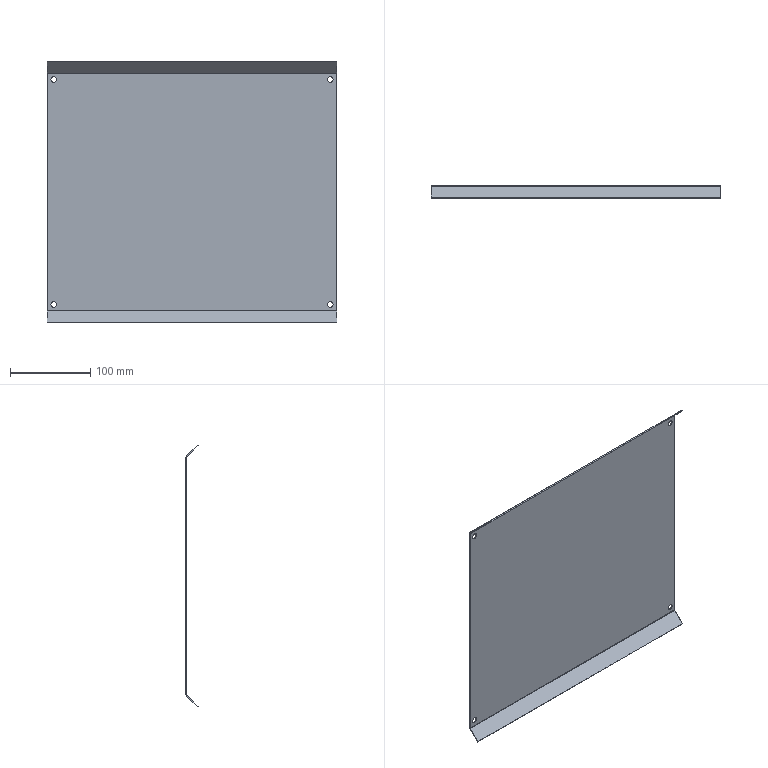Component | SolidWorks | CCD15ChainCover-1 | 1 solid | 30 faces | box 360 x 14.99 x 325.88 mm | volume 145179 mm3 | plane 18 | cylinder 12 | commonest cylinder face diameters 7 x8 3.873 x2 1.473 x2
STEP:
#1=CARTESIAN_POINT('',(-11.245,5.6,6.496));
#2=VERTEX_POINT('',#1);
#3=CARTESIAN_POINT('',(-11.521,5.6,6.496));
#4=VERTEX_POINT('',#3);
#5=CARTESIAN_POINT('',(-11.383,5.6,6.496));
#6=DIRECTION('',(0.,-1.,-0.));
#7=DIRECTION('',(-1.,-0.,-0.));
#8=AXIS2_PLACEMENT_3D('',#5,#6,#7);
#9=CIRCLE('',#8,0.1378);
#10=EDGE_CURVE('',#2,#4,#9,.T.);
#11=ORIENTED_EDGE('',*,*,#10,.T.);
#12=CARTESIAN_POINT('',(-11.521,5.648,6.496));
#13=VERTEX_POINT('',#12);
#14=CARTESIAN_POINT('',(-11.521,5.254,6.496));
#15=DIRECTION('',(-0.,1.,0.));
#16=VECTOR('',#15,39.37);
#17=LINE('',#14,#16);
#18=EDGE_CURVE('',#4,#13,#17,.T.);
#19=ORIENTED_EDGE('',*,*,#18,.T.);
#20=CARTESIAN_POINT('',(-11.245,5.648,6.496));
#21=VERTEX_POINT('',#20);
#22=CARTESIAN_POINT('',(-11.383,5.648,6.496));
#23=DIRECTION('',(-0.,1.,0.));
#24=DIRECTION('',(1.,0.,0.));
#25=AXIS2_PLACEMENT_3D('',#22,#23,#24);
#26=CIRCLE('',#25,0.1378);
#27=EDGE_CURVE('',#13,#21,#26,.T.);
#28=ORIENTED_EDGE('',*,*,#27,.T.);
#29=CARTESIAN_POINT('',(-11.245,5.254,6.496));
#30=DIRECTION('',(-0.,1.,0.));
#31=VECTOR('',#30,39.37);
#32=LINE('',#29,#31);
#33=EDGE_CURVE('',#2,#21,#32,.T.);
#34=ORIENTED_EDGE('',*,*,#33,.F.);
#35=EDGE_LOOP('',(#11,#19,#28,#34));
#36=FACE_OUTER_BOUND('',#35,.T.);
#37=CARTESIAN_POINT('',(-11.383,5.254,6.496));
#38=DIRECTION('',(-0.,1.,0.));
#39=DIRECTION('',(1.,0.,0.));
#40=AXIS2_PLACEMENT_3D('',#37,#38,#39);
#41=CYLINDRICAL_SURFACE('',#40,0.1378);
#42=ADVANCED_FACE('',(#36),#41,.F.);
#43=CARTESIAN_POINT('',(2.298,5.6,6.496));
#44=VERTEX_POINT('',#43);
#45=CARTESIAN_POINT('',(2.023,5.6,6.496));
#46=VERTEX_POINT('',#45);
#47=CARTESIAN_POINT('',(2.161,5.6,6.496));
#48=DIRECTION('',(0.,-1.,-0.));
#49=DIRECTION('',(-1.,-0.,-0.));
#50=AXIS2_PLACEMENT_3D('',#47,#48,#49);
#51=CIRCLE('',#50,0.1378);
#52=EDGE_CURVE('',#44,#46,#51,.T.);
#53=ORIENTED_EDGE('',*,*,#52,.T.);
#54=CARTESIAN_POINT('',(2.023,5.648,6.496));
#55=VERTEX_POINT('',#54);
#56=CARTESIAN_POINT('',(2.023,5.254,6.496));
#57=DIRECTION('',(-0.,1.,0.));
#58=VECTOR('',#57,39.37);
#59=LINE('',#56,#58);
#60=EDGE_CURVE('',#46,#55,#59,.T.);
#61=ORIENTED_EDGE('',*,*,#60,.T.);
#62=CARTESIAN_POINT('',(2.298,5.648,6.496));
#63=VERTEX_POINT('',#62);
#64=CARTESIAN_POINT('',(2.161,5.648,6.496));
#65=DIRECTION('',(-0.,1.,0.));
#66=DIRECTION('',(1.,0.,0.));
#67=AXIS2_PLACEMENT_3D('',#64,#65,#66);
#68=CIRCLE('',#67,0.1378);
#69=EDGE_CURVE('',#55,#63,#68,.T.);
#70=ORIENTED_EDGE('',*,*,#69,.T.);
#71=CARTESIAN_POINT('',(2.298,5.254,6.496));
#72=DIRECTION('',(-0.,1.,0.));
#73=VECTOR('',#72,39.37);
#74=LINE('',#71,#73);
#75=EDGE_CURVE('',#44,#63,#74,.T.);
#76=ORIENTED_EDGE('',*,*,#75,.F.);
#77=EDGE_LOOP('',(#53,#61,#70,#76));
#78=FACE_OUTER_BOUND('',#77,.T.);
#79=CARTESIAN_POINT('',(2.161,5.254,6.496));
#80=DIRECTION('',(-0.,1.,0.));
#81=DIRECTION('',(1.,0.,0.));
#82=AXIS2_PLACEMENT_3D('',#79,#80,#81);
#83=CYLINDRICAL_SURFACE('',#82,0.1378);
#84=ADVANCED_FACE('',(#78),#83,.F.);
#85=CARTESIAN_POINT('',(2.298,5.6,-4.528));
#86=VERTEX_POINT('',#85);
#87=CARTESIAN_POINT('',(2.023,5.6,-4.528));
#88=VERTEX_POINT('',#87);
#89=CARTESIAN_POINT('',(2.161,5.6,-4.528));
#90=DIRECTION('',(0.,-1.,-0.));
#91=DIRECTION('',(-1.,-0.,-0.));
#92=AXIS2_PLACEMENT_3D('',#89,#90,#91);
#93=CIRCLE('',#92,0.1378);
#94=EDGE_CURVE('',#86,#88,#93,.T.);
#95=ORIENTED_EDGE('',*,*,#94,.T.);
#96=CARTESIAN_POINT('',(2.023,5.648,-4.528));
#97=VERTEX_POINT('',#96);
#98=CARTESIAN_POINT('',(2.023,5.254,-4.528));
#99=DIRECTION('',(-0.,1.,0.));
#100=VECTOR('',#99,39.37);
#101=LINE('',#98,#100);
#102=EDGE_CURVE('',#88,#97,#101,.T.);
#103=ORIENTED_EDGE('',*,*,#102,.T.);
#104=CARTESIAN_POINT('',(2.298,5.648,-4.528));
#105=VERTEX_POINT('',#104);
#106=CARTESIAN_POINT('',(2.161,5.648,-4.528));
#107=DIRECTION('',(-0.,1.,0.));
#108=DIRECTION('',(1.,0.,0.));
#109=AXIS2_PLACEMENT_3D('',#106,#107,#108);
#110=CIRCLE('',#109,0.1378);
#111=EDGE_CURVE('',#97,#105,#110,.T.);
#112=ORIENTED_EDGE('',*,*,#111,.T.);
#113=CARTESIAN_POINT('',(2.298,5.254,-4.528));
#114=DIRECTION('',(-0.,1.,0.));
#115=VECTOR('',#114,39.37);
#116=LINE('',#113,#115);
#117=EDGE_CURVE('',#86,#105,#116,.T.);
#118=ORIENTED_EDGE('',*,*,#117,.F.);
#119=EDGE_LOOP('',(#95,#103,#112,#118));
#120=FACE_OUTER_BOUND('',#119,.T.);
#121=CARTESIAN_POINT('',(2.161,5.254,-4.528));
#122=DIRECTION('',(-0.,1.,0.));
#123=DIRECTION('',(1.,0.,0.));
#124=AXIS2_PLACEMENT_3D('',#121,#122,#123);
#125=CYLINDRICAL_SURFACE('',#124,0.1378);
#126=ADVANCED_FACE('',(#120),#125,.F.);
#127=CARTESIAN_POINT('',(-11.245,5.6,-4.528));
#128=VERTEX_POINT('',#127);
#129=CARTESIAN_POINT('',(-11.521,5.6,-4.528));
#130=VERTEX_POINT('',#129);
#131=CARTESIAN_POINT('',(-11.383,5.6,-4.528));
#132=DIRECTION('',(0.,-1.,-0.));
#133=DIRECTION('',(-1.,-0.,-0.));
#134=AXIS2_PLACEMENT_3D('',#131,#132,#133);
#135=CIRCLE('',#134,0.1378);
#136=EDGE_CURVE('',#128,#130,#135,.T.);
#137=ORIENTED_EDGE('',*,*,#136,.T.);
#138=CARTESIAN_POINT('',(-11.521,5.648,-4.528));
#139=VERTEX_POINT('',#138);
#140=CARTESIAN_POINT('',(-11.521,5.254,-4.528));
#141=DIRECTION('',(-0.,1.,0.));
#142=VECTOR('',#141,39.37);
#143=LINE('',#140,#142);
#144=EDGE_CURVE('',#130,#139,#143,.T.);
#145=ORIENTED_EDGE('',*,*,#144,.T.);
#146=CARTESIAN_POINT('',(-11.245,5.648,-4.528));
#147=VERTEX_POINT('',#146);
#148=CARTESIAN_POINT('',(-11.383,5.648,-4.528));
#149=DIRECTION('',(-0.,1.,0.));
#150=DIRECTION('',(1.,0.,0.));
#151=AXIS2_PLACEMENT_3D('',#148,#149,#150);
#152=CIRCLE('',#151,0.1378);
#153=EDGE_CURVE('',#139,#147,#152,.T.);
#154=ORIENTED_EDGE('',*,*,#153,.T.);
#155=CARTESIAN_POINT('',(-11.245,5.254,-4.528));
#156=DIRECTION('',(-0.,1.,0.));
#157=VECTOR('',#156,39.37);
#158=LINE('',#155,#157);
#159=EDGE_CURVE('',#128,#147,#158,.T.);
#160=ORIENTED_EDGE('',*,*,#159,.F.);
#161=EDGE_LOOP('',(#137,#145,#154,#160));
#162=FACE_OUTER_BOUND('',#161,.T.);
#163=CARTESIAN_POINT('',(-11.383,5.254,-4.528));
#164=DIRECTION('',(-0.,1.,0.));
#165=DIRECTION('',(1.,0.,0.));
#166=AXIS2_PLACEMENT_3D('',#163,#164,#165);
#167=CYLINDRICAL_SURFACE('',#166,0.1378);
#168=ADVANCED_FACE('',(#162),#167,.F.);
#169=ORIENTED_EDGE('',*,*,#10,.F.);
#170=CARTESIAN_POINT('',(-11.383,5.6,6.496));
#171=DIRECTION('',(0.,-1.,-0.));
#172=DIRECTION('',(-1.,-0.,-0.));
#173=AXIS2_PLACEMENT_3D('',#170,#171,#172);
#174=CIRCLE('',#173,0.1378);
#175=EDGE_CURVE('',#4,#2,#174,.T.);
#176=ORIENTED_EDGE('',*,*,#175,.F.);
#177=EDGE_LOOP('',(#169,#176));
#178=FACE_BOUND('',#177,.T.);
#179=ORIENTED_EDGE('',*,*,#52,.F.);
#180=CARTESIAN_POINT('',(2.161,5.6,6.496));
#181=DIRECTION('',(0.,-1.,-0.));
#182=DIRECTION('',(-1.,-0.,-0.));
#183=AXIS2_PLACEMENT_3D('',#180,#181,#182);
#184=CIRCLE('',#183,0.1378);
#185=EDGE_CURVE('',#46,#44,#184,.T.);
#186=ORIENTED_EDGE('',*,*,#185,.F.);
#187=EDGE_LOOP('',(#179,#186));
#188=FACE_BOUND('',#187,.T.);
#189=ORIENTED_EDGE('',*,*,#94,.F.);
#190=CARTESIAN_POINT('',(2.161,5.6,-4.528));
#191=DIRECTION('',(0.,-1.,-0.));
#192=DIRECTION('',(-1.,-0.,-0.));
#193=AXIS2_PLACEMENT_3D('',#190,#191,#192);
#194=CIRCLE('',#193,0.1378);
#195=EDGE_CURVE('',#88,#86,#194,.T.);
#196=ORIENTED_EDGE('',*,*,#195,.F.);
#197=EDGE_LOOP('',(#189,#196));
#198=FACE_BOUND('',#197,.T.);
#199=ORIENTED_EDGE('',*,*,#136,.F.);
#200=CARTESIAN_POINT('',(-11.383,5.6,-4.528));
#201=DIRECTION('',(0.,-1.,-0.));
#202=DIRECTION('',(-1.,-0.,-0.));
#203=AXIS2_PLACEMENT_3D('',#200,#201,#202);
#204=CIRCLE('',#203,0.1378);
#205=EDGE_CURVE('',#130,#128,#204,.T.);
#206=ORIENTED_EDGE('',*,*,#205,.F.);
#207=EDGE_LOOP('',(#199,#206));
#208=FACE_BOUND('',#207,.T.);
#209=CARTESIAN_POINT('',(2.476,5.6,6.811));
#210=VERTEX_POINT('',#209);
#211=CARTESIAN_POINT('',(2.476,5.6,-4.842));
#212=VERTEX_POINT('',#211);
#213=CARTESIAN_POINT('',(2.476,5.6,6.89));
#214=DIRECTION('',(0.,0.,-1.));
#215=VECTOR('',#214,39.37);
#216=LINE('',#213,#215);
#217=EDGE_CURVE('',#210,#212,#216,.T.);
#218=ORIENTED_EDGE('',*,*,#217,.F.);
#219=CARTESIAN_POINT('',(-11.698,5.6,6.811));
#220=VERTEX_POINT('',#219);
#221=CARTESIAN_POINT('',(-11.698,5.6,6.811));
#222=DIRECTION('',(1.,0.,0.));
#223=VECTOR('',#222,39.37);
#224=LINE('',#221,#223);
#225=EDGE_CURVE('',#220,#210,#224,.T.);
#226=ORIENTED_EDGE('',*,*,#225,.F.);
#227=CARTESIAN_POINT('',(-11.698,5.6,-4.842));
#228=VERTEX_POINT('',#227);
#229=CARTESIAN_POINT('',(-11.698,5.6,6.89));
#230=DIRECTION('',(-0.,-0.,1.));
#231=VECTOR('',#230,39.37);
#232=LINE('',#229,#231);
#233=EDGE_CURVE('',#228,#220,#232,.T.);
#234=ORIENTED_EDGE('',*,*,#233,.F.);
#235=CARTESIAN_POINT('',(2.476,5.6,-4.842));
#236=DIRECTION('',(-1.,-0.,-0.));
#237=VECTOR('',#236,39.37);
#238=LINE('',#235,#237);
#239=EDGE_CURVE('',#212,#228,#238,.T.);
#240=ORIENTED_EDGE('',*,*,#239,.F.);
#241=EDGE_LOOP('',(#218,#226,#234,#240));
#242=FACE_OUTER_BOUND('',#241,.T.);
#243=CARTESIAN_POINT('',(-11.698,5.6,6.89));
#244=DIRECTION('',(0.,-1.,-0.));
#245=DIRECTION('',(-1.,-0.,-0.));
#246=AXIS2_PLACEMENT_3D('',#243,#244,#245);
#247=PLANE('',#246);
#248=ADVANCED_FACE('',(#178,#188,#198,#208,#242),#247,.T.);
#249=CARTESIAN_POINT('',(-11.383,5.648,6.496));
#250=DIRECTION('',(-0.,1.,0.));
#251=DIRECTION('',(1.,0.,0.));
#252=AXIS2_PLACEMENT_3D('',#249,#250,#251);
#253=CIRCLE('',#252,0.1378);
#254=EDGE_CURVE('',#21,#13,#253,.T.);
#255=ORIENTED_EDGE('',*,*,#254,.F.);
#256=ORIENTED_EDGE('',*,*,#27,.F.);
#257=EDGE_LOOP('',(#255,#256));
#258=FACE_BOUND('',#257,.T.);
#259=CARTESIAN_POINT('',(2.161,5.648,6.496));
#260=DIRECTION('',(-0.,1.,0.));
#261=DIRECTION('',(1.,0.,0.));
#262=AXIS2_PLACEMENT_3D('',#259,#260,#261);
#263=CIRCLE('',#262,0.1378);
#264=EDGE_CURVE('',#63,#55,#263,.T.);
#265=ORIENTED_EDGE('',*,*,#264,.F.);
#266=ORIENTED_EDGE('',*,*,#69,.F.);
#267=EDGE_LOOP('',(#265,#266));
#268=FACE_BOUND('',#267,.T.);
#269=CARTESIAN_POINT('',(2.161,5.648,-4.528));
#270=DIRECTION('',(-0.,1.,0.));
#271=DIRECTION('',(1.,0.,0.));
#272=AXIS2_PLACEMENT_3D('',#269,#270,#271);
#273=CIRCLE('',#272,0.1378);
#274=EDGE_CURVE('',#105,#97,#273,.T.);
#275=ORIENTED_EDGE('',*,*,#274,.F.);
#276=ORIENTED_EDGE('',*,*,#111,.F.);
#277=EDGE_LOOP('',(#275,#276));
#278=FACE_BOUND('',#277,.T.);
#279=CARTESIAN_POINT('',(-11.383,5.648,-4.528));
#280=DIRECTION('',(-0.,1.,0.));
#281=DIRECTION('',(1.,0.,0.));
#282=AXIS2_PLACEMENT_3D('',#279,#280,#281);
#283=CIRCLE('',#282,0.1378);
#284=EDGE_CURVE('',#147,#139,#283,.T.);
#285=ORIENTED_EDGE('',*,*,#284,.F.);
#286=ORIENTED_EDGE('',*,*,#153,.F.);
#287=EDGE_LOOP('',(#285,#286));
#288=FACE_BOUND('',#287,.T.);
#289=CARTESIAN_POINT('',(-11.698,5.648,6.811));
#290=VERTEX_POINT('',#289);
#291=CARTESIAN_POINT('',(2.476,5.648,6.811));
#292=VERTEX_POINT('',#291);
#293=CARTESIAN_POINT('',(-11.698,5.648,6.811));
#294=DIRECTION('',(1.,0.,0.));
#295=VECTOR('',#294,39.37);
#296=LINE('',#293,#295);
#297=EDGE_CURVE('',#290,#292,#296,.T.);
#298=ORIENTED_EDGE('',*,*,#297,.T.);
#299=CARTESIAN_POINT('',(2.476,5.648,-4.842));
#300=VERTEX_POINT('',#299);
#301=CARTESIAN_POINT('',(2.476,5.648,6.89));
#302=DIRECTION('',(0.,0.,-1.));
#303=VECTOR('',#302,39.37);
#304=LINE('',#301,#303);
#305=EDGE_CURVE('',#292,#300,#304,.T.);
#306=ORIENTED_EDGE('',*,*,#305,.T.);
#307=CARTESIAN_POINT('',(-11.698,5.648,-4.842));
#308=VERTEX_POINT('',#307);
#309=CARTESIAN_POINT('',(2.476,5.648,-4.842));
#310=DIRECTION('',(-1.,-0.,-0.));
#311=VECTOR('',#310,39.37);
#312=LINE('',#309,#311);
#313=EDGE_CURVE('',#300,#308,#312,.T.);
#314=ORIENTED_EDGE('',*,*,#313,.T.);
#315=CARTESIAN_POINT('',(-11.698,5.648,6.89));
#316=DIRECTION('',(-0.,-0.,1.));
#317=VECTOR('',#316,39.37);
#318=LINE('',#315,#317);
#319=EDGE_CURVE('',#308,#290,#318,.T.);
#320=ORIENTED_EDGE('',*,*,#319,.T.);
#321=EDGE_LOOP('',(#298,#306,#314,#320));
#322=FACE_OUTER_BOUND('',#321,.T.);
#323=CARTESIAN_POINT('',(-11.698,5.648,6.89));
#324=DIRECTION('',(0.,-1.,-0.));
#325=DIRECTION('',(-1.,-0.,-0.));
#326=AXIS2_PLACEMENT_3D('',#323,#324,#325);
#327=PLANE('',#326);
#328=ADVANCED_FACE('',(#258,#268,#278,#288,#322),#327,.F.);
#329=ORIENTED_EDGE('',*,*,#233,.T.);
#330=CARTESIAN_POINT('',(-11.698,5.6,6.811));
#331=DIRECTION('',(-0.,1.,0.));
#332=VECTOR('',#331,39.37);
#333=LINE('',#330,#332);
#334=EDGE_CURVE('',#220,#290,#333,.T.);
#335=ORIENTED_EDGE('',*,*,#334,.T.);
#336=ORIENTED_EDGE('',*,*,#319,.F.);
#337=CARTESIAN_POINT('',(-11.698,5.6,-4.842));
#338=DIRECTION('',(-0.,1.,0.));
#339=VECTOR('',#338,39.37);
#340=LINE('',#337,#339);
#341=EDGE_CURVE('',#228,#308,#340,.T.);
#342=ORIENTED_EDGE('',*,*,#341,.F.);
#343=EDGE_LOOP('',(#329,#335,#336,#342));
#344=FACE_OUTER_BOUND('',#343,.T.);
#345=CARTESIAN_POINT('',(-11.698,5.6,6.89));
#346=DIRECTION('',(-1.,-0.,-0.));
#347=DIRECTION('',(-0.,1.,0.));
#348=AXIS2_PLACEMENT_3D('',#345,#346,#347);
#349=PLANE('',#348);
#350=ADVANCED_FACE('',(#344),#349,.T.);
#351=CARTESIAN_POINT('',(2.476,5.6,6.811));
#352=DIRECTION('',(-0.,1.,0.));
#353=VECTOR('',#352,39.37);
#354=LINE('',#351,#353);
#355=EDGE_CURVE('',#210,#292,#354,.T.);
#356=ORIENTED_EDGE('',*,*,#355,.F.);
#357=ORIENTED_EDGE('',*,*,#217,.T.);
#358=CARTESIAN_POINT('',(2.476,5.6,-4.842));
#359=DIRECTION('',(-0.,1.,0.));
#360=VECTOR('',#359,39.37);
#361=LINE('',#358,#360);
#362=EDGE_CURVE('',#212,#300,#361,.T.);
#363=ORIENTED_EDGE('',*,*,#362,.T.);
#364=ORIENTED_EDGE('',*,*,#305,.F.);
#365=EDGE_LOOP('',(#356,#357,#363,#364));
#366=FACE_OUTER_BOUND('',#365,.T.);
#367=CARTESIAN_POINT('',(2.476,5.6,6.89));
#368=DIRECTION('',(1.,0.,0.));
#369=DIRECTION('',(0.,-1.,-0.));
#370=AXIS2_PLACEMENT_3D('',#367,#368,#369);
#371=PLANE('',#370);
#372=ADVANCED_FACE('',(#366),#371,.T.);
#373=CARTESIAN_POINT('',(-11.698,5.592,-4.863));
#374=VERTEX_POINT('',#373);
#375=CARTESIAN_POINT('',(-11.698,5.625,-4.896));
#376=VERTEX_POINT('',#375);
#377=CARTESIAN_POINT('',(-11.698,5.625,-4.896));
#378=DIRECTION('',(-0.,0.7071,-0.7071));
#379=VECTOR('',#378,39.37);
#380=LINE('',#377,#379);
#381=EDGE_CURVE('',#374,#376,#380,.T.);
#382=ORIENTED_EDGE('',*,*,#381,.F.);
#383=CARTESIAN_POINT('',(-11.698,5.571,-4.842));
#384=DIRECTION('',(-1.,-0.,-0.));
#385=DIRECTION('',(0.,-1.,0.));
#386=AXIS2_PLACEMENT_3D('',#383,#384,#385);
#387=CIRCLE('',#386,0.029);
#388=EDGE_CURVE('',#228,#374,#387,.T.);
#389=ORIENTED_EDGE('',*,*,#388,.F.);
#390=ORIENTED_EDGE('',*,*,#341,.T.);
#391=CARTESIAN_POINT('',(-11.698,5.571,-4.842));
#392=DIRECTION('',(-1.,-0.,-0.));
#393=DIRECTION('',(0.,-1.,-0.));
#394=AXIS2_PLACEMENT_3D('',#391,#392,#393);
#395=CIRCLE('',#394,0.07624);
#396=EDGE_CURVE('',#308,#376,#395,.T.);
#397=ORIENTED_EDGE('',*,*,#396,.T.);
#398=EDGE_LOOP('',(#382,#389,#390,#397));
#399=FACE_OUTER_BOUND('',#398,.T.);
#400=CARTESIAN_POINT('',(-11.698,5.571,-4.842));
#401=DIRECTION('',(-1.,-0.,-0.));
#402=DIRECTION('',(-0.,1.,0.));
#403=AXIS2_PLACEMENT_3D('',#400,#401,#402);
#404=PLANE('',#403);
#405=ADVANCED_FACE('',(#399),#404,.T.);
#406=CARTESIAN_POINT('',(2.476,5.592,-4.863));
#407=VERTEX_POINT('',#406);
#408=CARTESIAN_POINT('',(2.476,5.571,-4.842));
#409=DIRECTION('',(1.,0.,0.));
#410=DIRECTION('',(0.,-1.,0.));
#411=AXIS2_PLACEMENT_3D('',#408,#409,#410);
#412=CIRCLE('',#411,0.029);
#413=EDGE_CURVE('',#407,#212,#412,.T.);
#414=ORIENTED_EDGE('',*,*,#413,.F.);
#415=CARTESIAN_POINT('',(2.476,5.625,-4.896));
#416=VERTEX_POINT('',#415);
#417=CARTESIAN_POINT('',(2.476,5.592,-4.863));
#418=DIRECTION('',(-0.,0.7071,-0.7071));
#419=VECTOR('',#418,39.37);
#420=LINE('',#417,#419);
#421=EDGE_CURVE('',#407,#416,#420,.T.);
#422=ORIENTED_EDGE('',*,*,#421,.T.);
#423=CARTESIAN_POINT('',(2.476,5.571,-4.842));
#424=DIRECTION('',(1.,0.,0.));
#425=DIRECTION('',(0.,-1.,0.));
#426=AXIS2_PLACEMENT_3D('',#423,#424,#425);
#427=CIRCLE('',#426,0.07624);
#428=EDGE_CURVE('',#416,#300,#427,.T.);
#429=ORIENTED_EDGE('',*,*,#428,.T.);
#430=ORIENTED_EDGE('',*,*,#362,.F.);
#431=EDGE_LOOP('',(#414,#422,#429,#430));
#432=FACE_OUTER_BOUND('',#431,.T.);
#433=CARTESIAN_POINT('',(2.476,5.571,-4.842));
#434=DIRECTION('',(-1.,-0.,-0.));
#435=DIRECTION('',(-0.,1.,0.));
#436=AXIS2_PLACEMENT_3D('',#433,#434,#435);
#437=PLANE('',#436);
#438=ADVANCED_FACE('',(#432),#437,.F.);
#439=ORIENTED_EDGE('',*,*,#313,.F.);
#440=ORIENTED_EDGE('',*,*,#428,.F.);
#441=CARTESIAN_POINT('',(-11.698,5.625,-4.896));
#442=DIRECTION('',(-1.,-0.,-0.));
#443=VECTOR('',#442,39.37);
#444=LINE('',#441,#443);
#445=EDGE_CURVE('',#416,#376,#444,.T.);
#446=ORIENTED_EDGE('',*,*,#445,.T.);
#447=ORIENTED_EDGE('',*,*,#396,.F.);
#448=EDGE_LOOP('',(#439,#440,#446,#447));
#449=FACE_OUTER_BOUND('',#448,.T.);
#450=CARTESIAN_POINT('',(2.476,5.571,-4.842));
#451=DIRECTION('',(1.,0.,0.));
#452=DIRECTION('',(0.,0.7071,-0.7071));
#453=AXIS2_PLACEMENT_3D('',#450,#451,#452);
#454=CYLINDRICAL_SURFACE('',#453,0.07624);
#455=ADVANCED_FACE('',(#449),#454,.T.);
#456=ORIENTED_EDGE('',*,*,#239,.T.);
#457=ORIENTED_EDGE('',*,*,#388,.T.);
#458=CARTESIAN_POINT('',(-11.698,5.592,-4.863));
#459=DIRECTION('',(1.,0.,0.));
#460=VECTOR('',#459,39.37);
#461=LINE('',#458,#460);
#462=EDGE_CURVE('',#374,#407,#461,.T.);
#463=ORIENTED_EDGE('',*,*,#462,.T.);
#464=ORIENTED_EDGE('',*,*,#413,.T.);
#465=EDGE_LOOP('',(#456,#457,#463,#464));
#466=FACE_OUTER_BOUND('',#465,.T.);
#467=CARTESIAN_POINT('',(2.476,5.571,-4.842));
#468=DIRECTION('',(1.,0.,0.));
#469=DIRECTION('',(0.,0.7071,-0.7071));
#470=AXIS2_PLACEMENT_3D('',#467,#468,#469);
#471=CYLINDRICAL_SURFACE('',#470,0.029);
#472=ADVANCED_FACE('',(#466),#471,.F.);
#473=ORIENTED_EDGE('',*,*,#421,.F.);
#474=CARTESIAN_POINT('',(2.476,5.058,-5.397));
#475=VERTEX_POINT('',#474);
#476=CARTESIAN_POINT('',(2.476,5.058,-5.397));
#477=DIRECTION('',(0.,-0.7071,-0.7071));
#478=VECTOR('',#477,39.37);
#479=LINE('',#476,#478);
#480=EDGE_CURVE('',#407,#475,#479,.T.);
#481=ORIENTED_EDGE('',*,*,#480,.T.);
#482=CARTESIAN_POINT('',(2.476,5.091,-5.431));
#483=VERTEX_POINT('',#482);
#484=CARTESIAN_POINT('',(2.476,5.091,-5.431));
#485=DIRECTION('',(0.,-0.7071,0.7071));
#486=VECTOR('',#485,39.37);
#487=LINE('',#484,#486);
#488=EDGE_CURVE('',#483,#475,#487,.T.);
#489=ORIENTED_EDGE('',*,*,#488,.F.);
#490=CARTESIAN_POINT('',(2.476,11.563,1.041));
#491=DIRECTION('',(0.,-0.7071,-0.7071));
#492=VECTOR('',#491,39.37);
#493=LINE('',#490,#492);
#494=EDGE_CURVE('',#416,#483,#493,.T.);
#495=ORIENTED_EDGE('',*,*,#494,.F.);
#496=EDGE_LOOP('',(#473,#481,#489,#495));
#497=FACE_OUTER_BOUND('',#496,.T.);
#498=CARTESIAN_POINT('',(2.476,5.091,-5.431));
#499=DIRECTION('',(-1.,-0.,-0.));
#500=DIRECTION('',(-0.,1.,0.));
#501=AXIS2_PLACEMENT_3D('',#498,#499,#500);
#502=PLANE('',#501);
#503=ADVANCED_FACE('',(#497),#502,.F.);
#504=ORIENTED_EDGE('',*,*,#381,.T.);
#505=CARTESIAN_POINT('',(-11.698,5.091,-5.431));
#506=VERTEX_POINT('',#505);
#507=CARTESIAN_POINT('',(-11.698,11.563,1.041));
#508=DIRECTION('',(-0.,0.7071,0.7071));
#509=VECTOR('',#508,39.37);
#510=LINE('',#507,#509);
#511=EDGE_CURVE('',#506,#376,#510,.T.);
#512=ORIENTED_EDGE('',*,*,#511,.F.);
#513=CARTESIAN_POINT('',(-11.698,5.058,-5.397));
#514=VERTEX_POINT('',#513);
#515=CARTESIAN_POINT('',(-11.698,5.091,-5.431));
#516=DIRECTION('',(0.,-0.7071,0.7071));
#517=VECTOR('',#516,39.37);
#518=LINE('',#515,#517);
#519=EDGE_CURVE('',#506,#514,#518,.T.);
#520=ORIENTED_EDGE('',*,*,#519,.T.);
#521=CARTESIAN_POINT('',(-11.698,5.6,-4.854));
#522=DIRECTION('',(-0.,0.7071,0.7071));
#523=VECTOR('',#522,39.37);
#524=LINE('',#521,#523);
#525=EDGE_CURVE('',#514,#374,#524,.T.);
#526=ORIENTED_EDGE('',*,*,#525,.T.);
#527=EDGE_LOOP('',(#504,#512,#520,#526));
#528=FACE_OUTER_BOUND('',#527,.T.);
#529=CARTESIAN_POINT('',(-11.698,5.634,-4.888));
#530=DIRECTION('',(1.,0.,0.));
#531=DIRECTION('',(0.,-1.,-0.));
#532=AXIS2_PLACEMENT_3D('',#529,#530,#531);
#533=PLANE('',#532);
#534=ADVANCED_FACE('',(#528),#533,.F.);
#535=ORIENTED_EDGE('',*,*,#445,.F.);
#536=ORIENTED_EDGE('',*,*,#494,.T.);
#537=CARTESIAN_POINT('',(-11.698,5.091,-5.431));
#538=DIRECTION('',(-1.,-0.,-0.));
#539=VECTOR('',#538,39.37);
#540=LINE('',#537,#539);
#541=EDGE_CURVE('',#483,#506,#540,.T.);
#542=ORIENTED_EDGE('',*,*,#541,.T.);
#543=ORIENTED_EDGE('',*,*,#511,.T.);
#544=EDGE_LOOP('',(#535,#536,#542,#543));
#545=FACE_OUTER_BOUND('',#544,.T.);
#546=CARTESIAN_POINT('',(-11.698,11.563,1.041));
#547=DIRECTION('',(0.,-0.7071,0.7071));
#548=DIRECTION('',(0.,-0.7071,-0.7071));
#549=AXIS2_PLACEMENT_3D('',#546,#547,#548);
#550=PLANE('',#549);
#551=ADVANCED_FACE('',(#545),#550,.F.);
#552=ORIENTED_EDGE('',*,*,#480,.F.);
#553=ORIENTED_EDGE('',*,*,#462,.F.);
#554=ORIENTED_EDGE('',*,*,#525,.F.);
#555=CARTESIAN_POINT('',(-11.698,5.058,-5.397));
#556=DIRECTION('',(-1.,-0.,-0.));
#557=VECTOR('',#556,39.37);
#558=LINE('',#555,#557);
#559=EDGE_CURVE('',#475,#514,#558,.T.);
#560=ORIENTED_EDGE('',*,*,#559,.F.);
#561=EDGE_LOOP('',(#552,#553,#554,#560));
#562=FACE_OUTER_BOUND('',#561,.T.);
#563=CARTESIAN_POINT('',(-11.698,11.53,1.075));
#564=DIRECTION('',(0.,-0.7071,0.7071));
#565=DIRECTION('',(0.,-0.7071,-0.7071));
#566=AXIS2_PLACEMENT_3D('',#563,#564,#565);
#567=PLANE('',#566);
#568=ADVANCED_FACE('',(#562),#567,.T.);
#569=ORIENTED_EDGE('',*,*,#559,.T.);
#570=ORIENTED_EDGE('',*,*,#519,.F.);
#571=ORIENTED_EDGE('',*,*,#541,.F.);
#572=ORIENTED_EDGE('',*,*,#488,.T.);
#573=EDGE_LOOP('',(#569,#570,#571,#572));
#574=FACE_OUTER_BOUND('',#573,.T.);
#575=CARTESIAN_POINT('',(-11.698,5.091,-5.431));
#576=DIRECTION('',(-0.,0.7071,0.7071));
#577=DIRECTION('',(0.,-0.7071,0.7071));
#578=AXIS2_PLACEMENT_3D('',#575,#576,#577);
#579=PLANE('',#578);
#580=ADVANCED_FACE('',(#574),#579,.F.);
#581=CARTESIAN_POINT('',(2.476,5.592,6.831));
#582=VERTEX_POINT('',#581);
#583=CARTESIAN_POINT('',(2.476,5.625,6.865));
#584=VERTEX_POINT('',#583);
#585=CARTESIAN_POINT('',(2.476,5.625,6.865));
#586=DIRECTION('',(-0.,0.7071,0.7071));
#587=VECTOR('',#586,39.37);
#588=LINE('',#585,#587);
#589=EDGE_CURVE('',#582,#584,#588,.T.);
#590=ORIENTED_EDGE('',*,*,#589,.F.);
#591=CARTESIAN_POINT('',(2.476,5.571,6.811));
#592=DIRECTION('',(1.,0.,0.));
#593=DIRECTION('',(0.,1.,0.));
#594=AXIS2_PLACEMENT_3D('',#591,#592,#593);
#595=CIRCLE('',#594,0.029);
#596=EDGE_CURVE('',#210,#582,#595,.T.);
#597=ORIENTED_EDGE('',*,*,#596,.F.);
#598=ORIENTED_EDGE('',*,*,#355,.T.);
#599=CARTESIAN_POINT('',(2.476,5.571,6.811));
#600=DIRECTION('',(1.,0.,0.));
#601=DIRECTION('',(-0.,1.,0.));
#602=AXIS2_PLACEMENT_3D('',#599,#600,#601);
#603=CIRCLE('',#602,0.07624);
#604=EDGE_CURVE('',#292,#584,#603,.T.);
#605=ORIENTED_EDGE('',*,*,#604,.T.);
#606=EDGE_LOOP('',(#590,#597,#598,#605));
#607=FACE_OUTER_BOUND('',#606,.T.);
#608=CARTESIAN_POINT('',(2.476,5.571,6.811));
#609=DIRECTION('',(1.,0.,0.));
#610=DIRECTION('',(0.,-1.,-0.));
#611=AXIS2_PLACEMENT_3D('',#608,#609,#610);
#612=PLANE('',#611);
#613=ADVANCED_FACE('',(#607),#612,.T.);
#614=CARTESIAN_POINT('',(-11.698,5.592,6.831));
#615=VERTEX_POINT('',#614);
#616=CARTESIAN_POINT('',(-11.698,5.571,6.811));
#617=DIRECTION('',(-1.,-0.,-0.));
#618=DIRECTION('',(0.,1.,0.));
#619=AXIS2_PLACEMENT_3D('',#616,#617,#618);
#620=CIRCLE('',#619,0.029);
#621=EDGE_CURVE('',#615,#220,#620,.T.);
#622=ORIENTED_EDGE('',*,*,#621,.F.);
#623=CARTESIAN_POINT('',(-11.698,5.625,6.865));
#624=VERTEX_POINT('',#623);
#625=CARTESIAN_POINT('',(-11.698,5.592,6.831));
#626=DIRECTION('',(-0.,0.7071,0.7071));
#627=VECTOR('',#626,39.37);
#628=LINE('',#625,#627);
#629=EDGE_CURVE('',#615,#624,#628,.T.);
#630=ORIENTED_EDGE('',*,*,#629,.T.);
#631=CARTESIAN_POINT('',(-11.698,5.571,6.811));
#632=DIRECTION('',(-1.,-0.,-0.));
#633=DIRECTION('',(0.,1.,0.));
#634=AXIS2_PLACEMENT_3D('',#631,#632,#633);
#635=CIRCLE('',#634,0.07624);
#636=EDGE_CURVE('',#624,#290,#635,.T.);
#637=ORIENTED_EDGE('',*,*,#636,.T.);
#638=ORIENTED_EDGE('',*,*,#334,.F.);
#639=EDGE_LOOP('',(#622,#630,#637,#638));
#640=FACE_OUTER_BOUND('',#639,.T.);
#641=CARTESIAN_POINT('',(-11.698,5.571,6.811));
#642=DIRECTION('',(1.,0.,0.));
#643=DIRECTION('',(0.,-1.,-0.));
#644=AXIS2_PLACEMENT_3D('',#641,#642,#643);
#645=PLANE('',#644);
#646=ADVANCED_FACE('',(#640),#645,.F.);
#647=ORIENTED_EDGE('',*,*,#297,.F.);
#648=ORIENTED_EDGE('',*,*,#636,.F.);
#649=CARTESIAN_POINT('',(2.476,5.625,6.865));
#650=DIRECTION('',(1.,0.,0.));
#651=VECTOR('',#650,39.37);
#652=LINE('',#649,#651);
#653=EDGE_CURVE('',#624,#584,#652,.T.);
#654=ORIENTED_EDGE('',*,*,#653,.T.);
#655=ORIENTED_EDGE('',*,*,#604,.F.);
#656=EDGE_LOOP('',(#647,#648,#654,#655));
#657=FACE_OUTER_BOUND('',#656,.T.);
#658=CARTESIAN_POINT('',(-11.698,5.571,6.811));
#659=DIRECTION('',(-1.,-0.,-0.));
#660=DIRECTION('',(0.,0.7071,0.7071));
#661=AXIS2_PLACEMENT_3D('',#658,#659,#660);
#662=CYLINDRICAL_SURFACE('',#661,0.07624);
#663=ADVANCED_FACE('',(#657),#662,.T.);
#664=ORIENTED_EDGE('',*,*,#225,.T.);
#665=ORIENTED_EDGE('',*,*,#596,.T.);
#666=CARTESIAN_POINT('',(2.476,5.592,6.831));
#667=DIRECTION('',(-1.,-0.,-0.));
#668=VECTOR('',#667,39.37);
#669=LINE('',#666,#668);
#670=EDGE_CURVE('',#582,#615,#669,.T.);
#671=ORIENTED_EDGE('',*,*,#670,.T.);
#672=ORIENTED_EDGE('',*,*,#621,.T.);
#673=EDGE_LOOP('',(#664,#665,#671,#672));
#674=FACE_OUTER_BOUND('',#673,.T.);
#675=CARTESIAN_POINT('',(-11.698,5.571,6.811));
#676=DIRECTION('',(-1.,-0.,-0.));
#677=DIRECTION('',(0.,0.7071,0.7071));
#678=AXIS2_PLACEMENT_3D('',#675,#676,#677);
#679=CYLINDRICAL_SURFACE('',#678,0.029);
#680=ADVANCED_FACE('',(#674),#679,.F.);
#681=ORIENTED_EDGE('',*,*,#629,.F.);
#682=CARTESIAN_POINT('',(-11.698,5.058,7.366));
#683=VERTEX_POINT('',#682);
#684=CARTESIAN_POINT('',(-11.698,5.058,7.366));
#685=DIRECTION('',(-0.,-0.7071,0.7071));
#686=VECTOR('',#685,39.37);
#687=LINE('',#684,#686);
#688=EDGE_CURVE('',#615,#683,#687,.T.);
#689=ORIENTED_EDGE('',*,*,#688,.T.);
#690=CARTESIAN_POINT('',(-11.698,5.091,7.399));
#691=VERTEX_POINT('',#690);
#692=CARTESIAN_POINT('',(-11.698,5.091,7.399));
#693=DIRECTION('',(0.,-0.7071,-0.7071));
#694=VECTOR('',#693,39.37);
#695=LINE('',#692,#694);
#696=EDGE_CURVE('',#691,#683,#695,.T.);
#697=ORIENTED_EDGE('',*,*,#696,.F.);
#698=CARTESIAN_POINT('',(-11.698,5.657,6.833));
#699=DIRECTION('',(-0.,-0.7071,0.7071));
#700=VECTOR('',#699,39.37);
#701=LINE('',#698,#700);
#702=EDGE_CURVE('',#624,#691,#701,.T.);
#703=ORIENTED_EDGE('',*,*,#702,.F.);
#704=EDGE_LOOP('',(#681,#689,#697,#703));
#705=FACE_OUTER_BOUND('',#704,.T.);
#706=CARTESIAN_POINT('',(-11.698,5.091,7.399));
#707=DIRECTION('',(1.,0.,0.));
#708=DIRECTION('',(0.,-1.,-0.));
#709=AXIS2_PLACEMENT_3D('',#706,#707,#708);
#710=PLANE('',#709);
#711=ADVANCED_FACE('',(#705),#710,.F.);
#712=ORIENTED_EDGE('',*,*,#589,.T.);
#713=CARTESIAN_POINT('',(2.476,5.091,7.399));
#714=VERTEX_POINT('',#713);
#715=CARTESIAN_POINT('',(2.476,5.657,6.833));
#716=DIRECTION('',(0.,0.7071,-0.7071));
#717=VECTOR('',#716,39.37);
#718=LINE('',#715,#717);
#719=EDGE_CURVE('',#714,#584,#718,.T.);
#720=ORIENTED_EDGE('',*,*,#719,.F.);
#721=CARTESIAN_POINT('',(2.476,5.058,7.366));
#722=VERTEX_POINT('',#721);
#723=CARTESIAN_POINT('',(2.476,5.091,7.399));
#724=DIRECTION('',(0.,-0.7071,-0.7071));
#725=VECTOR('',#724,39.37);
#726=LINE('',#723,#725);
#727=EDGE_CURVE('',#714,#722,#726,.T.);
#728=ORIENTED_EDGE('',*,*,#727,.T.);
#729=CARTESIAN_POINT('',(2.476,5.6,6.823));
#730=DIRECTION('',(0.,0.7071,-0.7071));
#731=VECTOR('',#730,39.37);
#732=LINE('',#729,#731);
#733=EDGE_CURVE('',#722,#582,#732,.T.);
#734=ORIENTED_EDGE('',*,*,#733,.T.);
#735=EDGE_LOOP('',(#712,#720,#728,#734));
#736=FACE_OUTER_BOUND('',#735,.T.);
#737=CARTESIAN_POINT('',(2.476,5.634,6.856));
#738=DIRECTION('',(-1.,-0.,-0.));
#739=DIRECTION('',(-0.,1.,0.));
#740=AXIS2_PLACEMENT_3D('',#737,#738,#739);
#741=PLANE('',#740);
#742=ADVANCED_FACE('',(#736),#741,.F.);
#743=ORIENTED_EDGE('',*,*,#653,.F.);
#744=ORIENTED_EDGE('',*,*,#702,.T.);
#745=CARTESIAN_POINT('',(-11.698,5.091,7.399));
#746=DIRECTION('',(1.,0.,0.));
#747=VECTOR('',#746,39.37);
#748=LINE('',#745,#747);
#749=EDGE_CURVE('',#691,#714,#748,.T.);
#750=ORIENTED_EDGE('',*,*,#749,.T.);
#751=ORIENTED_EDGE('',*,*,#719,.T.);
#752=EDGE_LOOP('',(#743,#744,#750,#751));
#753=FACE_OUTER_BOUND('',#752,.T.);
#754=CARTESIAN_POINT('',(-11.698,5.657,6.833));
#755=DIRECTION('',(0.,-0.7071,-0.7071));
#756=DIRECTION('',(0.,0.7071,-0.7071));
#757=AXIS2_PLACEMENT_3D('',#754,#755,#756);
#758=PLANE('',#757);
#759=ADVANCED_FACE('',(#753),#758,.F.);
#760=ORIENTED_EDGE('',*,*,#688,.F.);
#761=ORIENTED_EDGE('',*,*,#670,.F.);
#762=ORIENTED_EDGE('',*,*,#733,.F.);
#763=CARTESIAN_POINT('',(2.476,5.058,7.366));
#764=DIRECTION('',(1.,0.,0.));
#765=VECTOR('',#764,39.37);
#766=LINE('',#763,#765);
#767=EDGE_CURVE('',#683,#722,#766,.T.);
#768=ORIENTED_EDGE('',*,*,#767,.F.);
#769=EDGE_LOOP('',(#760,#761,#762,#768));
#770=FACE_OUTER_BOUND('',#769,.T.);
#771=CARTESIAN_POINT('',(-11.698,5.624,6.799));
#772=DIRECTION('',(0.,-0.7071,-0.7071));
#773=DIRECTION('',(0.,0.7071,-0.7071));
#774=AXIS2_PLACEMENT_3D('',#771,#772,#773);
#775=PLANE('',#774);
#776=ADVANCED_FACE('',(#770),#775,.T.);
#777=ORIENTED_EDGE('',*,*,#767,.T.);
#778=ORIENTED_EDGE('',*,*,#727,.F.);
#779=ORIENTED_EDGE('',*,*,#749,.F.);
#780=ORIENTED_EDGE('',*,*,#696,.T.);
#781=EDGE_LOOP('',(#777,#778,#779,#780));
#782=FACE_OUTER_BOUND('',#781,.T.);
#783=CARTESIAN_POINT('',(2.476,5.091,7.399));
#784=DIRECTION('',(0.,0.7071,-0.7071));
#785=DIRECTION('',(-0.,0.7071,0.7071));
#786=AXIS2_PLACEMENT_3D('',#783,#784,#785);
#787=PLANE('',#786);
#788=ADVANCED_FACE('',(#782),#787,.F.);
#789=ORIENTED_EDGE('',*,*,#144,.F.);
#790=ORIENTED_EDGE('',*,*,#205,.T.);
#791=ORIENTED_EDGE('',*,*,#159,.T.);
#792=ORIENTED_EDGE('',*,*,#284,.T.);
#793=EDGE_LOOP('',(#789,#790,#791,#792));
#794=FACE_OUTER_BOUND('',#793,.T.);
#795=CARTESIAN_POINT('',(-11.383,5.254,-4.528));
#796=DIRECTION('',(-0.,1.,0.));
#797=DIRECTION('',(1.,0.,0.));
#798=AXIS2_PLACEMENT_3D('',#795,#796,#797);
#799=CYLINDRICAL_SURFACE('',#798,0.1378);
#800=ADVANCED_FACE('',(#794),#799,.F.);
#801=ORIENTED_EDGE('',*,*,#102,.F.);
#802=ORIENTED_EDGE('',*,*,#195,.T.);
#803=ORIENTED_EDGE('',*,*,#117,.T.);
#804=ORIENTED_EDGE('',*,*,#274,.T.);
#805=EDGE_LOOP('',(#801,#802,#803,#804));
#806=FACE_OUTER_BOUND('',#805,.T.);
#807=CARTESIAN_POINT('',(2.161,5.254,-4.528));
#808=DIRECTION('',(-0.,1.,0.));
#809=DIRECTION('',(1.,0.,0.));
#810=AXIS2_PLACEMENT_3D('',#807,#808,#809);
#811=CYLINDRICAL_SURFACE('',#810,0.1378);
#812=ADVANCED_FACE('',(#806),#811,.F.);
#813=ORIENTED_EDGE('',*,*,#60,.F.);
#814=ORIENTED_EDGE('',*,*,#185,.T.);
#815=ORIENTED_EDGE('',*,*,#75,.T.);
#816=ORIENTED_EDGE('',*,*,#264,.T.);
#817=EDGE_LOOP('',(#813,#814,#815,#816));
#818=FACE_OUTER_BOUND('',#817,.T.);
#819=CARTESIAN_POINT('',(2.161,5.254,6.496));
#820=DIRECTION('',(-0.,1.,0.));
#821=DIRECTION('',(1.,0.,0.));
#822=AXIS2_PLACEMENT_3D('',#819,#820,#821);
#823=CYLINDRICAL_SURFACE('',#822,0.1378);
#824=ADVANCED_FACE('',(#818),#823,.F.);
#825=ORIENTED_EDGE('',*,*,#18,.F.);
#826=ORIENTED_EDGE('',*,*,#175,.T.);
#827=ORIENTED_EDGE('',*,*,#33,.T.);
#828=ORIENTED_EDGE('',*,*,#254,.T.);
#829=EDGE_LOOP('',(#825,#826,#827,#828));
#830=FACE_OUTER_BOUND('',#829,.T.);
#831=CARTESIAN_POINT('',(-11.383,5.254,6.496));
#832=DIRECTION('',(-0.,1.,0.));
#833=DIRECTION('',(1.,0.,0.));
#834=AXIS2_PLACEMENT_3D('',#831,#832,#833);
#835=CYLINDRICAL_SURFACE('',#834,0.1378);
#836=ADVANCED_FACE('',(#830),#835,.F.);
#837=CLOSED_SHELL('',(#42,#84,#126,#168,#248,#328,#350,#372,#405,#438,#455,#472,#503,#534,#551,#568,#580,#613,#646,#663,#680,#711,#742,#759,#776,#788,#800,#812,#824,#836));
#838=MANIFOLD_SOLID_BREP('',#837);
#839=CARTESIAN_POINT('',(0.,0.,0.));
#840=DIRECTION('',(0.,0.,1.));
#841=DIRECTION('',(1.,0.,0.));
#842=AXIS2_PLACEMENT_3D('',#839,#840,#841);
#843=(LENGTH_UNIT()NAMED_UNIT(*)SI_UNIT($,.METRE.));
#844=LENGTH_MEASURE_WITH_UNIT(LENGTH_MEASURE(0.0254),#843);
#845=DIMENSIONAL_EXPONENTS(1.,0.,0.,0.,0.,0.,0.);
#846=(CONVERSION_BASED_UNIT('',#844)LENGTH_UNIT()NAMED_UNIT(#845));
#847=UNCERTAINTY_MEASURE_WITH_UNIT(LENGTH_MEASURE(0.00001),#846,'','');
#848=(NAMED_UNIT(*)PLANE_ANGLE_UNIT()SI_UNIT($,.RADIAN.));
#849=(NAMED_UNIT(*)SI_UNIT($,.STERADIAN.)SOLID_ANGLE_UNIT());
#850=(GEOMETRIC_REPRESENTATION_CONTEXT(3)GLOBAL_UNCERTAINTY_ASSIGNED_CONTEXT((#847))GLOBAL_UNIT_ASSIGNED_CONTEXT((#846,#848,#849))REPRESENTATION_CONTEXT('',''));
#851=ADVANCED_BREP_SHAPE_REPRESENTATION('',(#838,#842),#850);
#852=COLOUR_RGB('',0.7922,0.8196,0.9333);
#853=FILL_AREA_STYLE_COLOUR('',#852);
#854=FILL_AREA_STYLE('',(#853));
#855=SURFACE_STYLE_FILL_AREA(#854);
#856=SURFACE_SIDE_STYLE('',(#855));
#857=SURFACE_STYLE_USAGE(.BOTH.,#856);
#858=PRESENTATION_STYLE_ASSIGNMENT((#857));
#859=STYLED_ITEM('',(#858),#838);
#860=PRESENTATION_LAYER_ASSIGNMENT('','',(#859));
#861=(LENGTH_UNIT()NAMED_UNIT(*)SI_UNIT($,.METRE.));
#862=LENGTH_MEASURE_WITH_UNIT(LENGTH_MEASURE(0.0254),#861);
#863=DIMENSIONAL_EXPONENTS(1.,0.,0.,0.,0.,0.,0.);
#864=(CONVERSION_BASED_UNIT('',#862)LENGTH_UNIT()NAMED_UNIT(#863));
#865=UNCERTAINTY_MEASURE_WITH_UNIT(LENGTH_MEASURE(0.00001),#864,'','');
#866=(NAMED_UNIT(*)PLANE_ANGLE_UNIT()SI_UNIT($,.RADIAN.));
#867=(NAMED_UNIT(*)SI_UNIT($,.STERADIAN.)SOLID_ANGLE_UNIT());
#868=(GEOMETRIC_REPRESENTATION_CONTEXT(3)GLOBAL_UNCERTAINTY_ASSIGNED_CONTEXT((#865))GLOBAL_UNIT_ASSIGNED_CONTEXT((#864,#866,#867))REPRESENTATION_CONTEXT('',''));
#869=MECHANICAL_DESIGN_GEOMETRIC_PRESENTATION_REPRESENTATION('',(#859),#868);